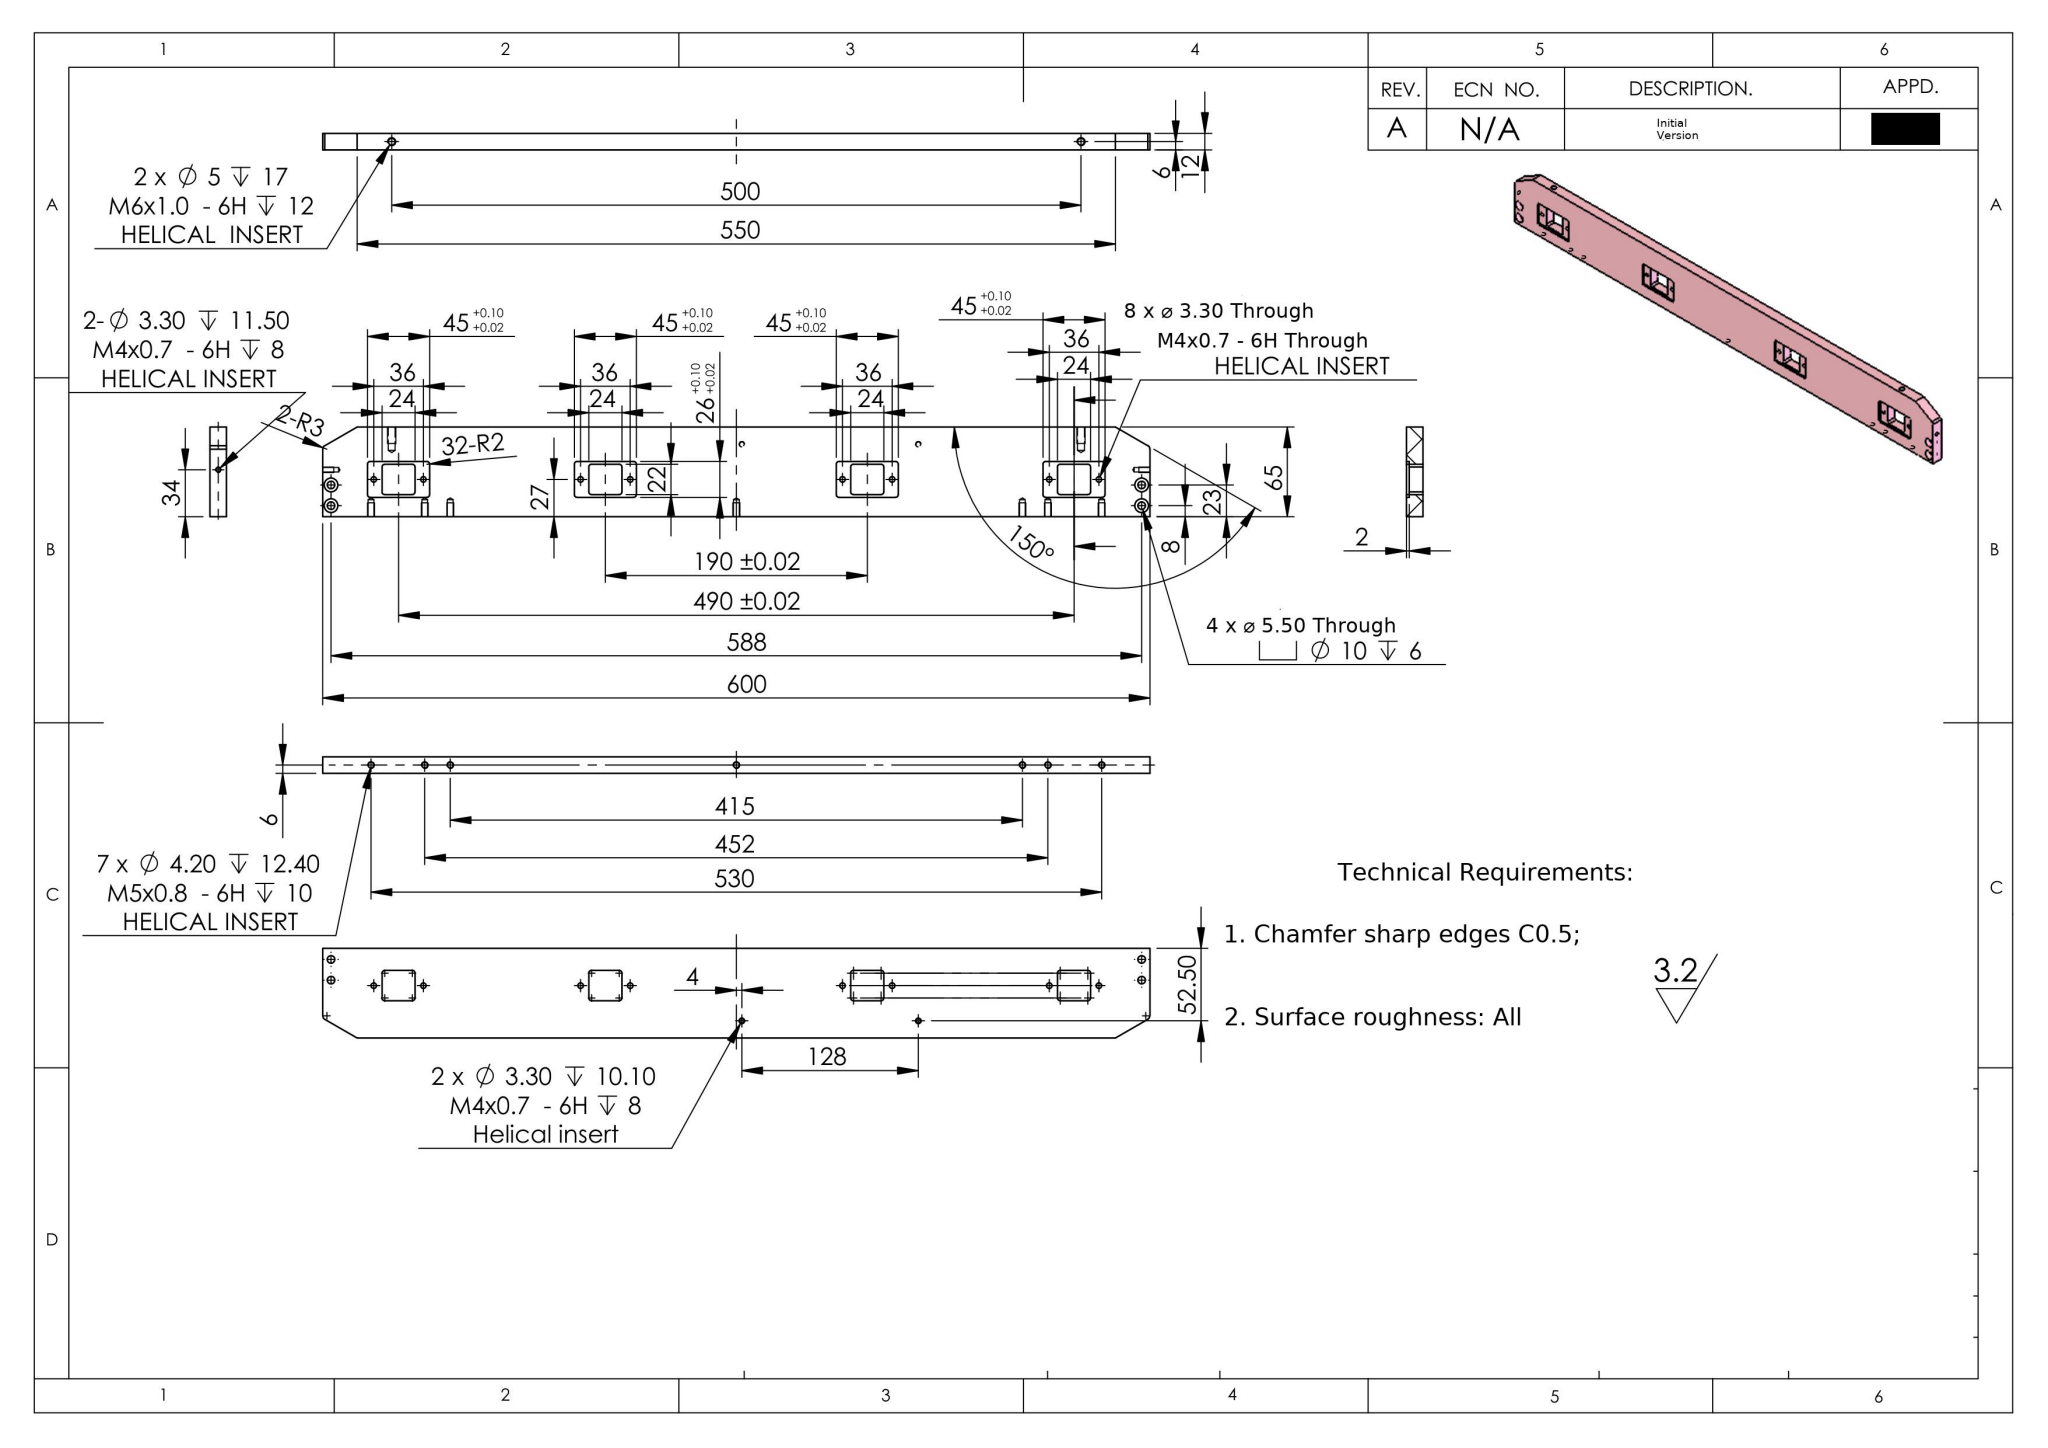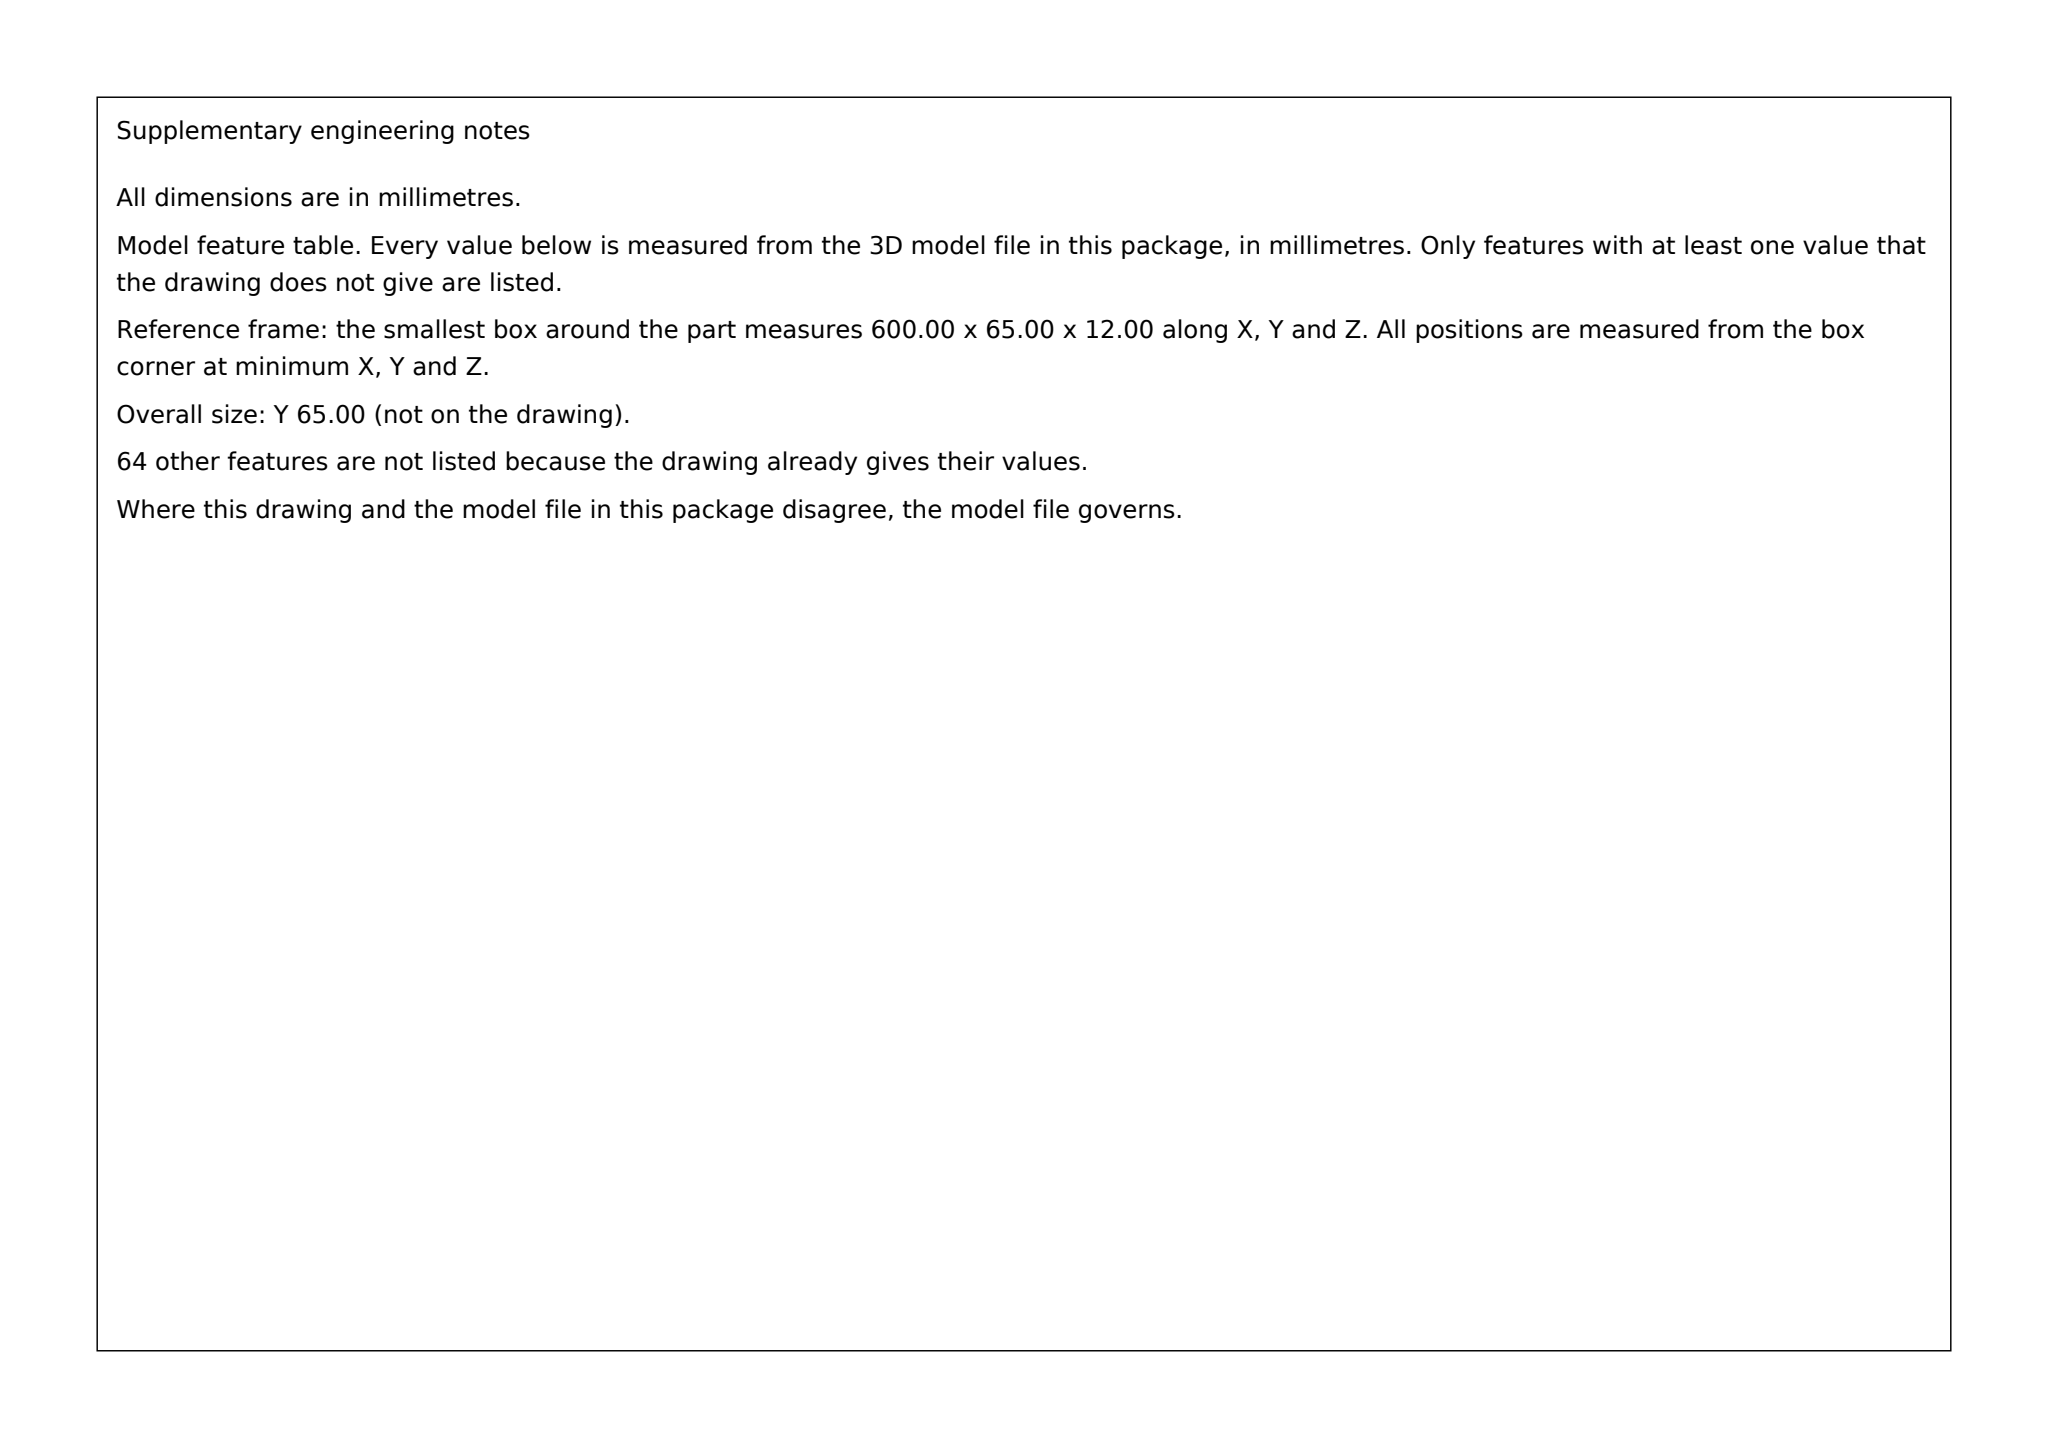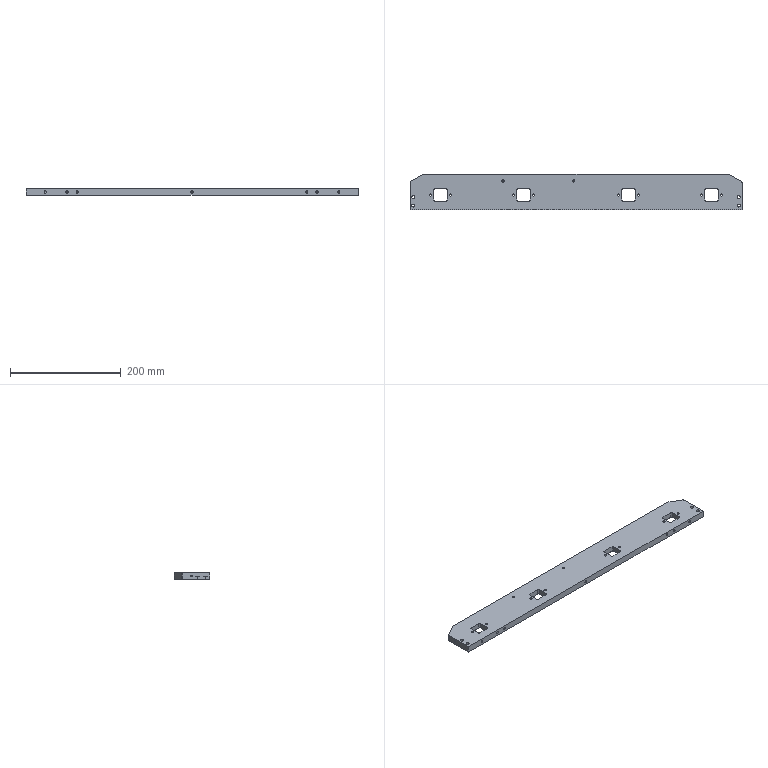Part | SolidWorks | mm | 1 solid | 172 faces | box 600 x 65 x 12 mm | volume 427507 mm3 | cylinder 96 | plane 50 | cone 26 | commonest cylinder face diameters 4 x52 4.2 x14 3.3 x8 5.5 x8 10 x8 5 x4 6 x2